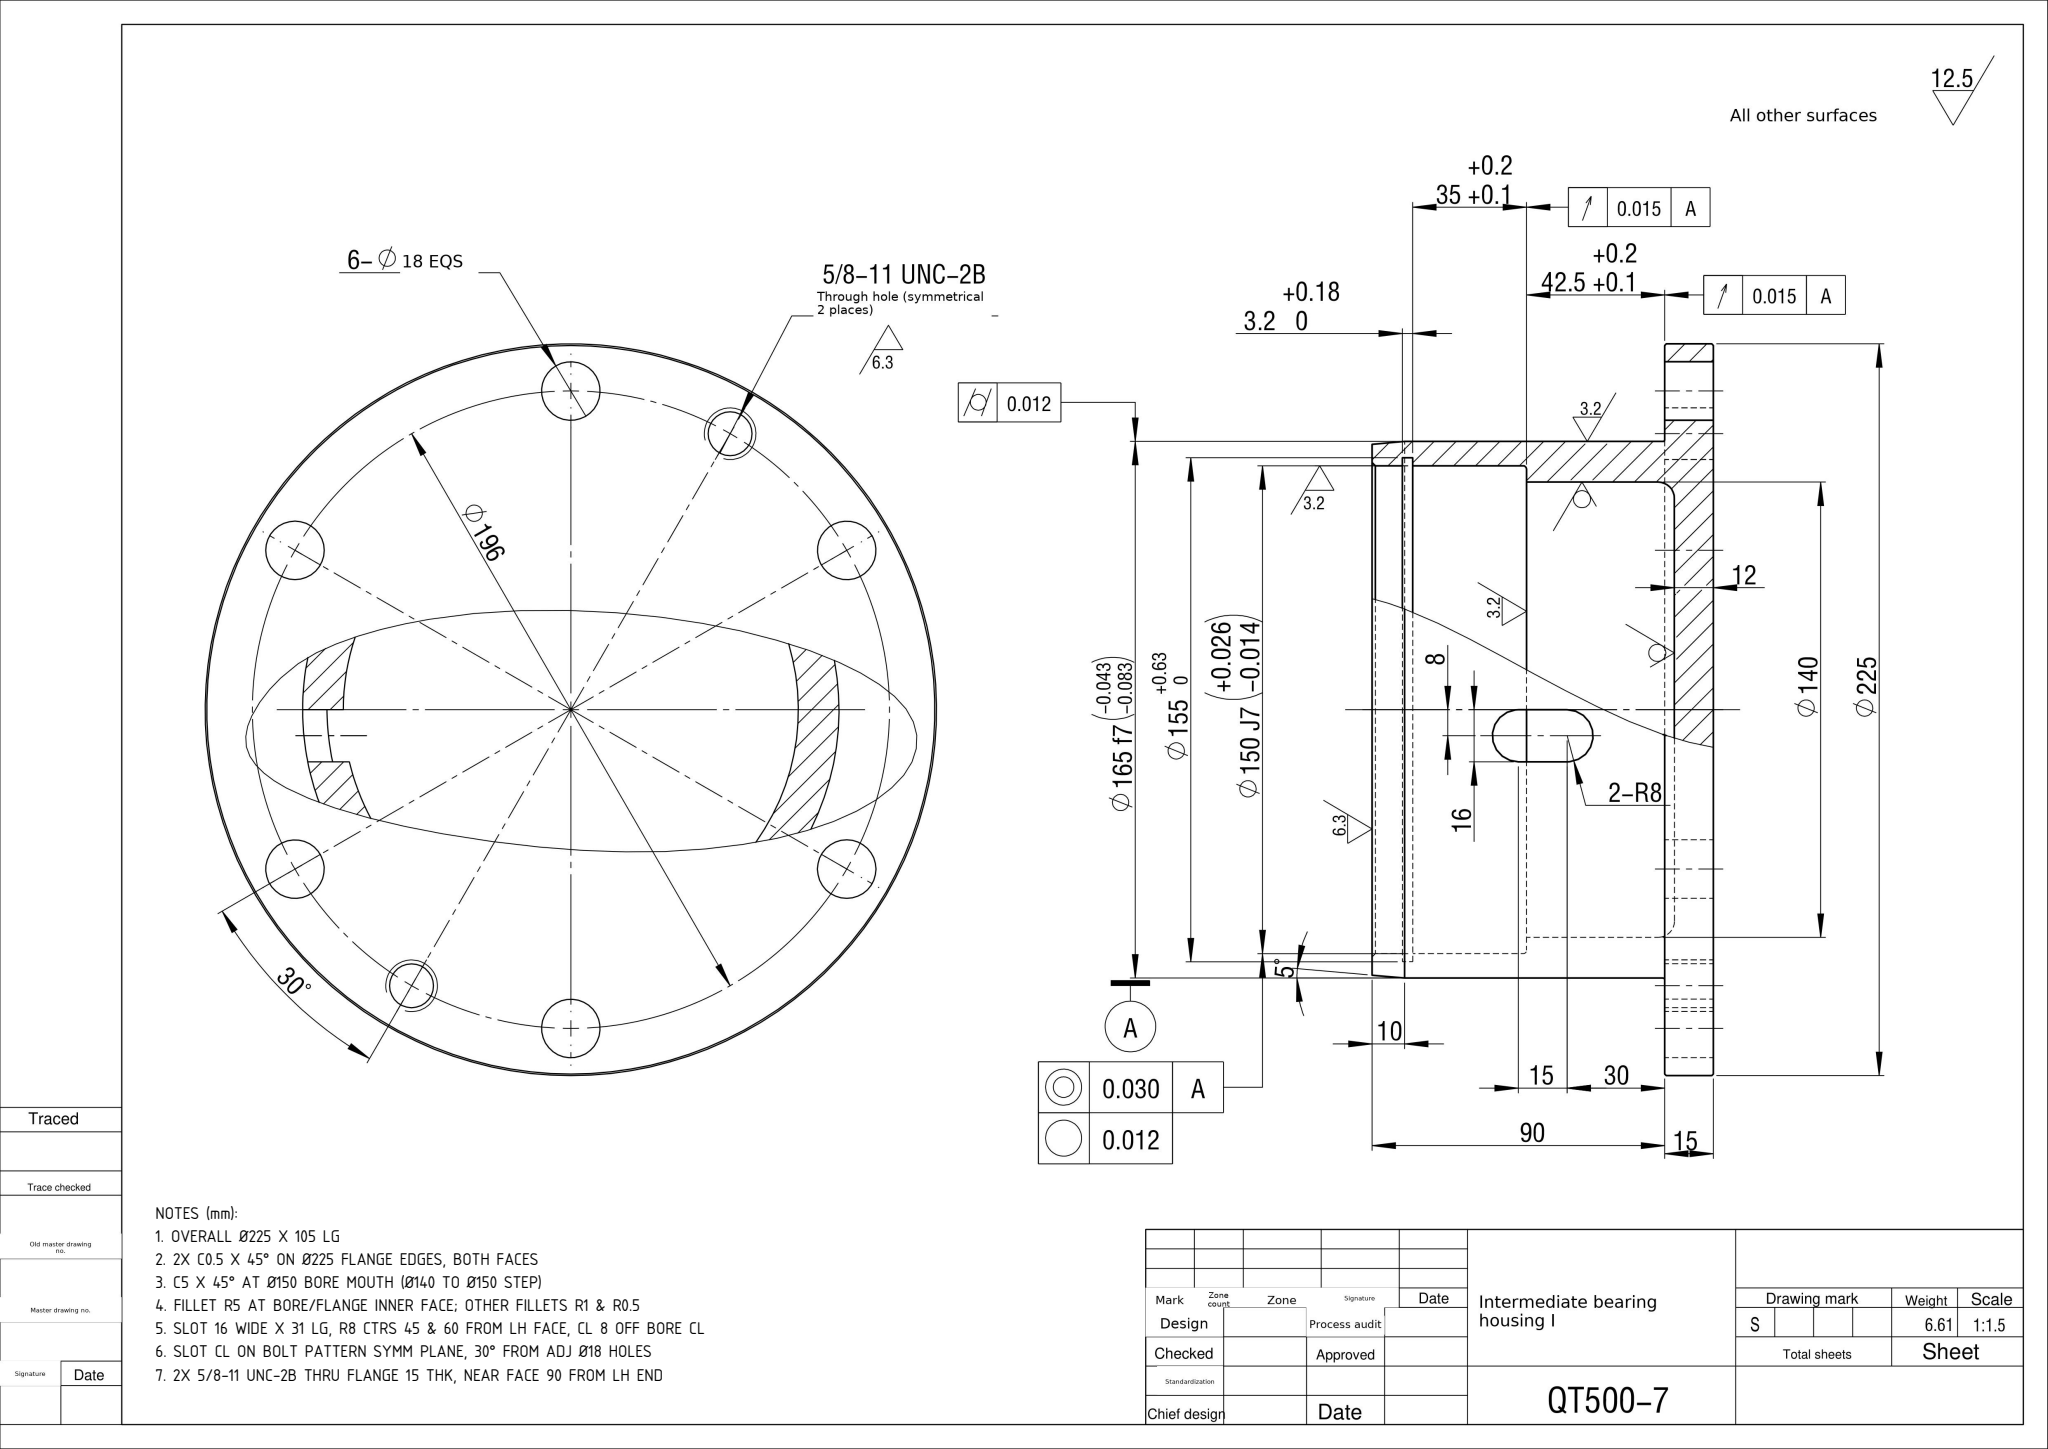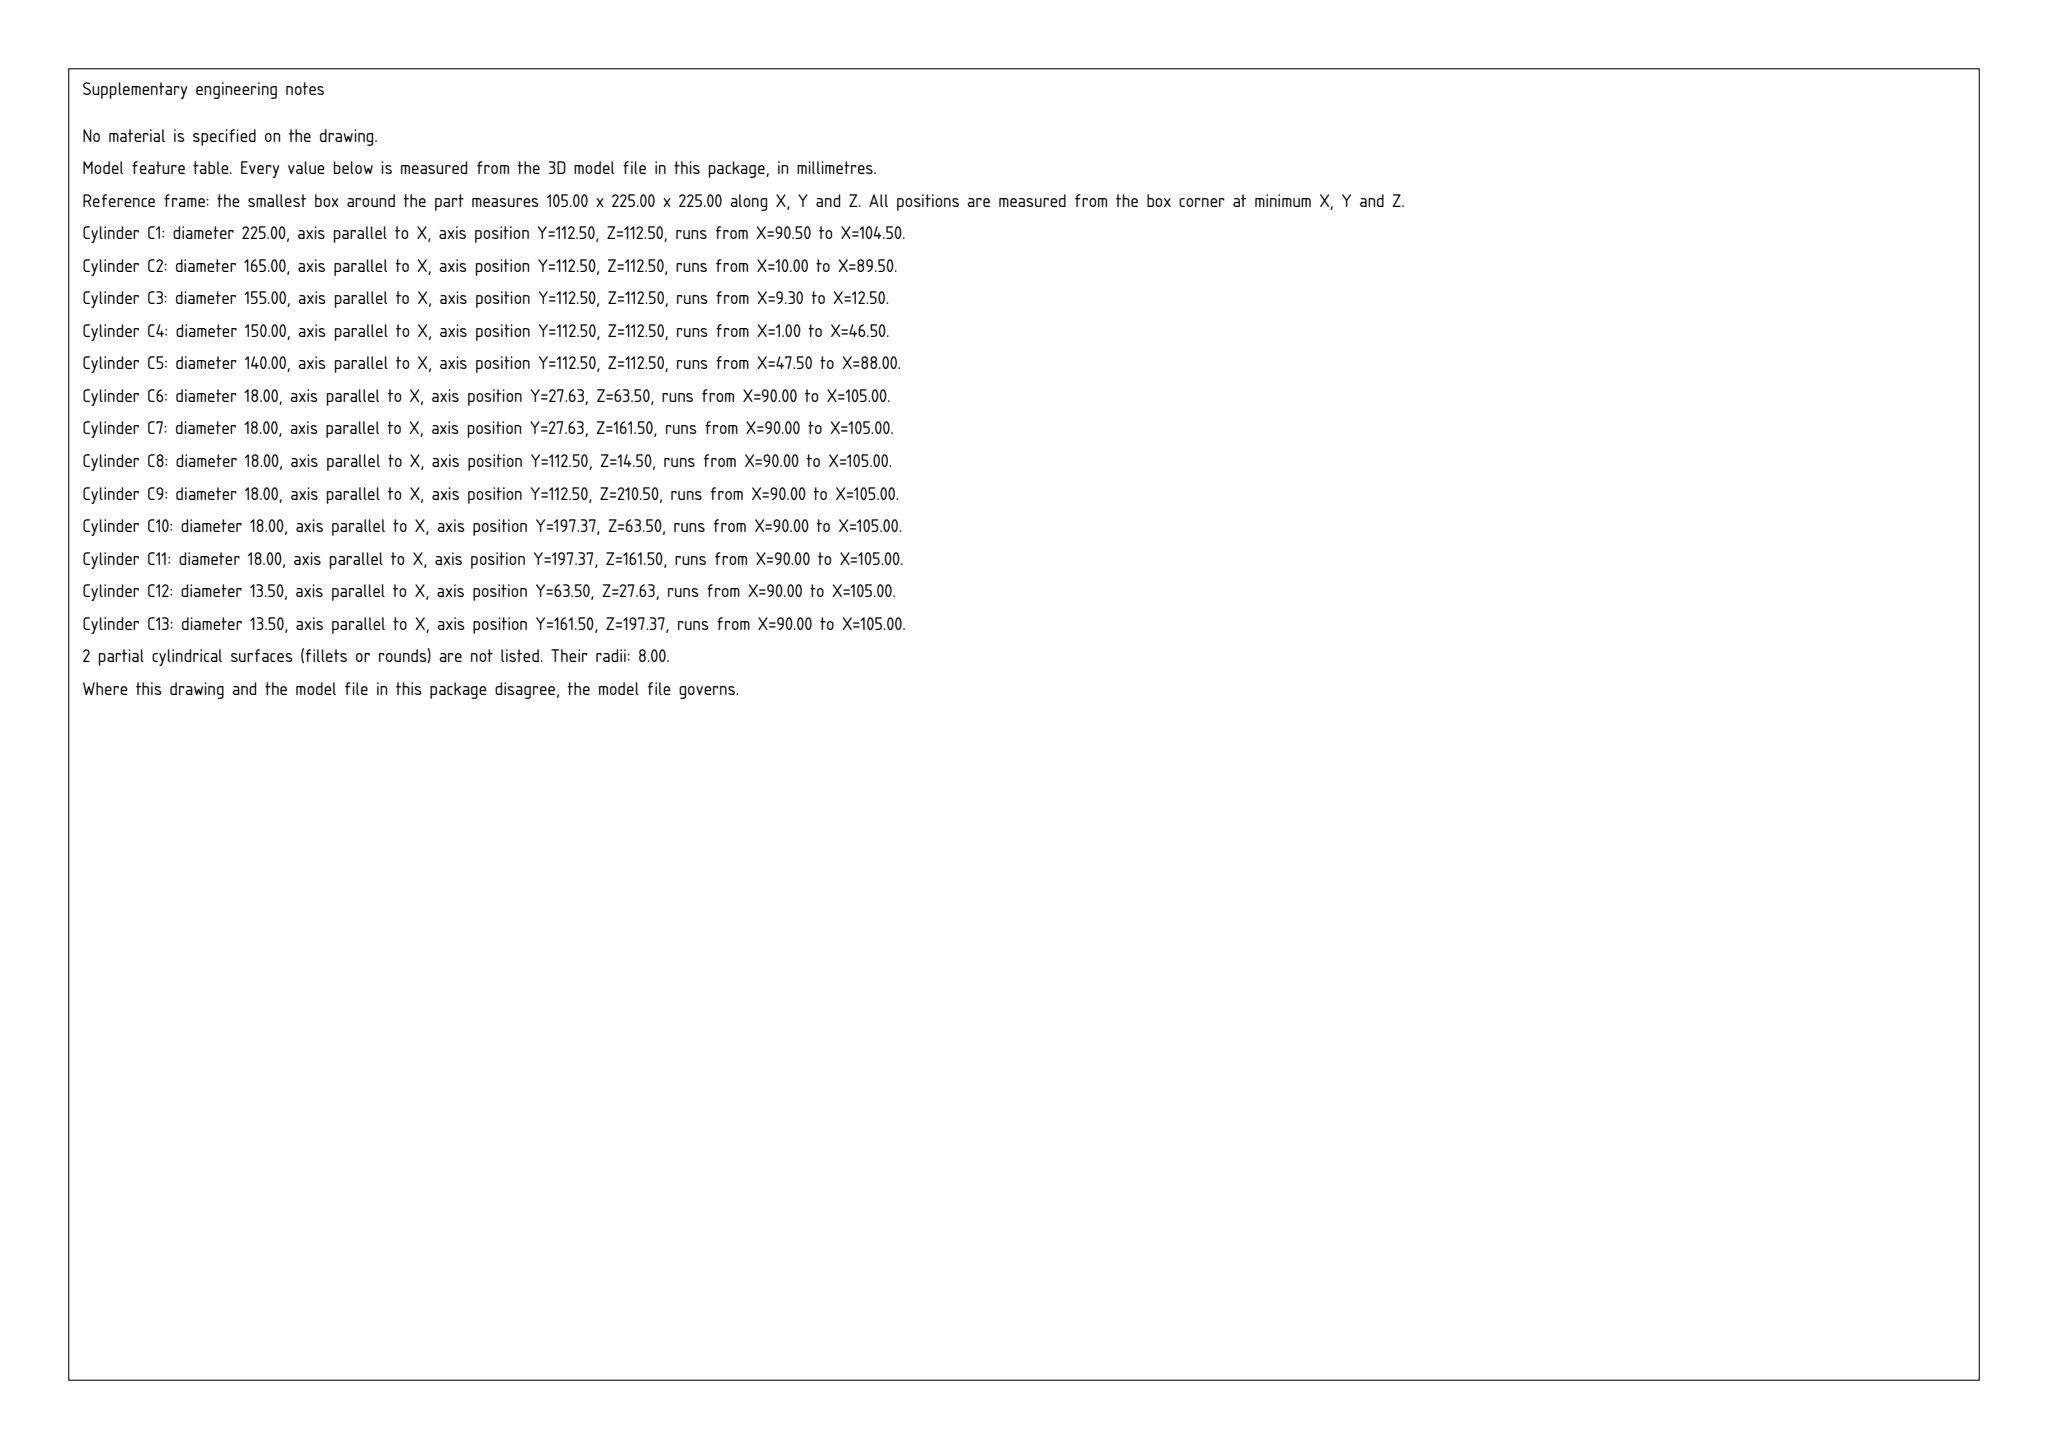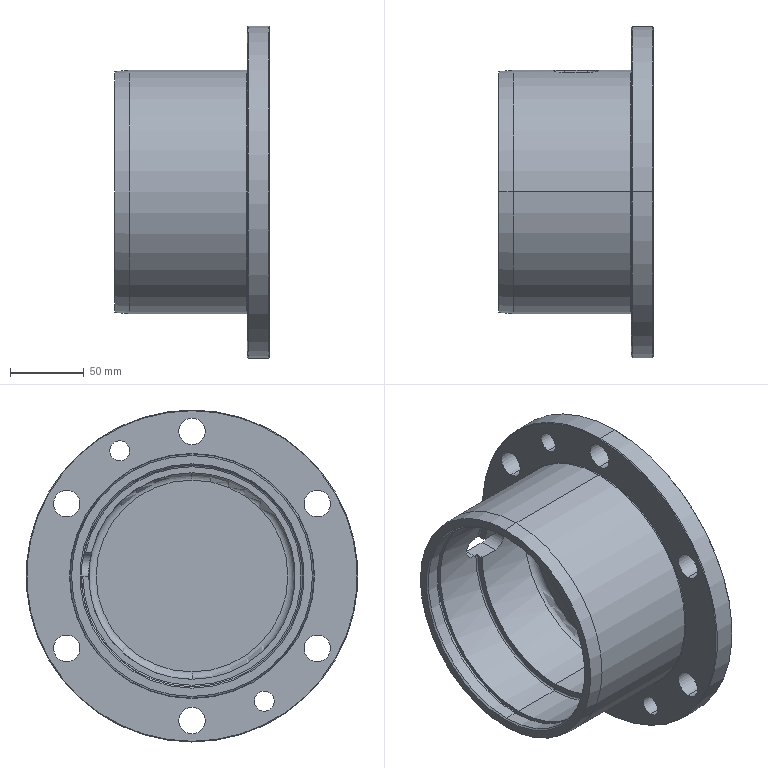Part | SolidWorks | mm | 1 solid | 54 faces | box 105 x 225 x 225 mm | volume 944926 mm3 | cylinder 30 | plane 9 | cone 8 | torus 7 | commonest cylinder face diameters 18 x12 13.492 x4 150 x4 155 x2 225 x2 140 x2 165 x2 16 x2
Drawing notes:
OVERALL Ø225 X 105 LG | from the solid: bbox 105 x 225 x 225; Ø225 flange cyl, x-planes 0.0 and 105.0
2X C0.5 X 45° ON Ø225 FLANGE EDGES, BOTH FACES | from the solid: cones 90° incl at ref dia 225 and 224 -> 0.5 radial drop
C5 X 45° AT Ø150 BORE MOUTH (Ø140 TO Ø150 STEP) | from the solid: cone 90° incl, ref dia 150 joining Ø140 & Ø150 bores
FILLET R5 AT BORE/FLANGE INNER FACE; OTHER FILLETS R1 & R0.5 | from the solid: fillet_radii [5.0 x2], [1.0 x3], [0.5 x2]
SLOT 16 WIDE X 31 LG, R8 CTRS 45 & 60 FROM LH FACE, CL 8 OFF BORE CL | from the solid: 16.0 dia cyls axis y at (x45,z120.5) & (x60,z120.5); 15 apart +16 = 31 OAL; bore axis z112.5, z-plane 128.5
SLOT CL ON BOLT PATTERN SYMM PLANE, 30° FROM ADJ Ø18 HOLES | from the solid: slot axis +Y from bore CL (112.5,112.5); Ø18 holes 30° each side of +Y
2X 5/8-11 UNC-2B THRU FLANGE 15 THK, NEAR FACE 90 FROM LH END | from the solid: 13.492 dia cyls axis x, len 15.0 at (y63.5,z27.63) & (y161.5,z197.37); x-planes 90.0 & 105.0; R98 BC
build123d program:
from build123d import *

# Parameters (mm, degrees)
FILLET6_R               = 1
CUT_EXTRUDE1_REACH      = 192.624
CUT_EXTRUDE1_END_RADIUS = 82.5
CHAMFER1_SIZE           = 1
SKETCH5_R               = 9
CUT_EXTRUDE3_DEPTH      = 50
CIRPATTERN1_COUNT       = 6
F_5_8_11_TAPPED_HOLE1_D = 13.492
CIRPATTERN2_COUNT       = 2
CHAMFER2_SIZE           = 0.5
FILLET4_R               = 5
FILLET5_R               = 0.5


with BuildPart() as part:
    # Sketch1 → Revolve1 (revolve)
    with BuildSketch(Plane.XY, mode=Mode.PRIVATE) as revolve1_sk:
        Polygon((0, 112.5), (-15, 112.5), (-15, 82.5), (-95, 82.5), (-105, 81.625), (-105, 75), (-95.7, 75), (-95.7, 77.5), (-92.5, 77.5), (-92.5, 75), (-57.5, 75), (-57.5, 70), (-12, 70), (-12, 0), (0, 0), align=None)
    revolve(revolve1_sk.sketch.rotate(Axis((-300.313, 0, 0), (1, 0, 0)), 90), axis=Axis((-300.313, 0, 0), (1, 0, 0)))

    # Fillet6
    fillet6_edges = [part.edges().sort_by_distance(p)[0] for p in [
        (-57.5, 0, -75),
    ]]
    fillet(fillet6_edges, radius=FILLET6_R)

    # Cut-Extrude1: up to this cylinder (the profile starts inside it)
    cut_extrude1_end = Plane(origin=(-52.5, 0, 0), z_dir=(-1, 0, 0)) * Cylinder(CUT_EXTRUDE1_END_RADIUS, 551.248, mode=Mode.PRIVATE)
    # Sketch2 → Cut-Extrude1 (cut, up to the surface)
    with BuildSketch(Plane(origin=(0, 0, 0), x_dir=(1, 0, 0), z_dir=(0, 1, 0)), mode=Mode.PRIVATE) as cut_extrude1_sk1:
        with BuildLine():
            Line((-60, 0), (-45, 0))
            ThreePointArc((-45, 0), (-37, -8), (-45, -16))
            Line((-45, -16), (-60, -16))
            ThreePointArc((-60, -16), (-68, -8), (-60, 0))
        make_face()
    cut_extrude1_tool1 = extrude(cut_extrude1_sk1.sketch, amount=CUT_EXTRUDE1_REACH, mode=Mode.PRIVATE) & cut_extrude1_end
    add(cut_extrude1_tool1.solids().sort_by_distance((-52.5, 0, 8))[0], mode=Mode.SUBTRACT)

    # Chamfer1
    chamfer1_edges = [part.edges().sort_by_distance(p)[0] for p in [
        (-105, 0, -75),
    ]]
    chamfer(chamfer1_edges, length=CHAMFER1_SIZE)

    # Sketch5 → Cut-Extrude3 (cut)
    with BuildSketch(Plane(origin=(0, 0, 0), x_dir=(0, 0, -1), z_dir=(1, 0, 0))):
        with Locations((49, 84.87)):
            Circle(SKETCH5_R)
    cut_extrude3 = extrude(amount=-CUT_EXTRUDE3_DEPTH, mode=Mode.SUBTRACT)

    # CirPattern1: Cut-Extrude3 ×6 about axis
    cirpattern1_axis = Axis((0, 0, 0), (1, 0, 0))
    for i in range(1, CIRPATTERN1_COUNT):
        add(cut_extrude3.rotate(cirpattern1_axis, i * 360 / CIRPATTERN1_COUNT), mode=Mode.SUBTRACT)

    # 5_8-11 Tapped Hole1 (through all)
    with Locations(Plane(origin=(0, -49, -84.87), x_dir=(0, 0, 1), z_dir=(1, 0, 0))):
        with Locations((0, 0)):
            f_5_8_11_tapped_hole1 = Hole(F_5_8_11_TAPPED_HOLE1_D / 2)

    # CirPattern2: 5_8-11 Tapped Hole1 ×2 about axis
    cirpattern2_axis = Axis((0, 0, 0), (1, 0, 0))
    for i in range(1, CIRPATTERN2_COUNT):
        add(f_5_8_11_tapped_hole1.rotate(cirpattern2_axis, i * 360 / CIRPATTERN2_COUNT), mode=Mode.SUBTRACT)

    # Chamfer2
    chamfer2_edges = [part.edges().sort_by_distance(p)[0] for p in [
        (-15, 0, -112.5),
        (0, 0, -112.5),
    ]]
    chamfer(chamfer2_edges, length=CHAMFER2_SIZE)

    # Fillet4
    fillet4_edges = [part.edges().sort_by_distance(p)[0] for p in [
        (-12, 0, -70),
    ]]
    fillet(fillet4_edges, radius=FILLET4_R)

    # Fillet5
    fillet5_edges = [part.edges().sort_by_distance(p)[0] for p in [
        (-15, 0, -82.5),
    ]]
    fillet(fillet5_edges, radius=FILLET5_R)


solid = part.part